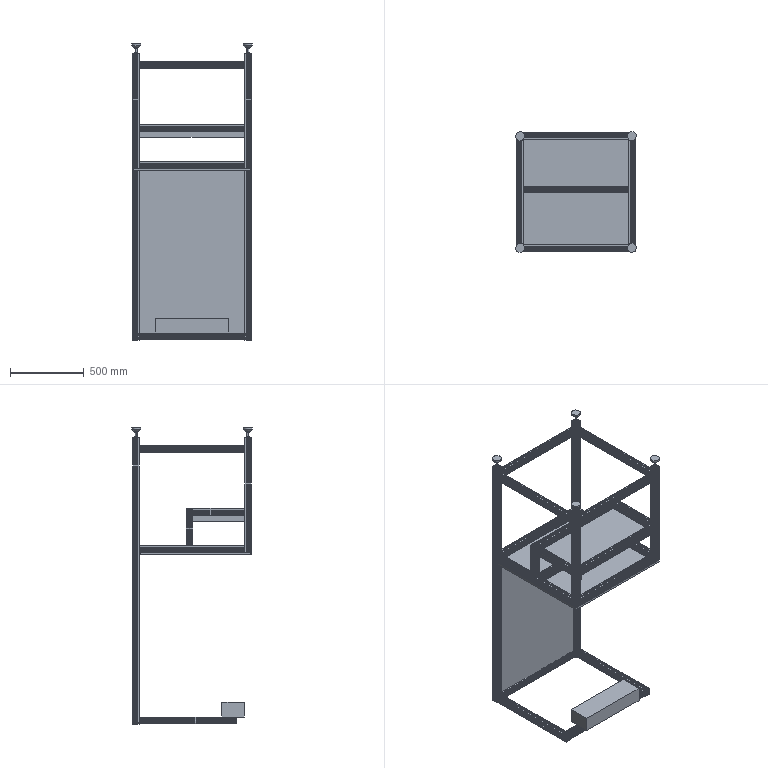Assembly | SolidWorks | mm | 41 component files | 41 solids | 3749 faces | box 815 x 815 x 2003 mm | volume 35568573 mm3 | plane 2366 | cylinder 1301 | cone 78 | spline 4 | commonest cylinder face diameters 2 x414 3 x276 1 x230 12.5 x145 6 x118 10 x36 2.5 x24 12 x16
Bill of materials:
dub02-B | 1 | Pine | Thin, nearly square flat plate with very small corner radii and no visible holes or other features.
FBR12nut | 4 |  | Hexagonal prism with a central round through-bore, with chamfered corners on both end faces. The shape is like a hex nut.
pad160_12_70pad1 | 4 |  | Part that turns around a single axis: a large circular disc with a short cylindrical rim and a conical taper underneath, a small hexagonal collar below the cone, and a long slender cylindrical shank with a chamfered end. The shape is like a leveling foot or swivel pad.
HFC8_4545_Bc | 6 |  | Square plate with rounded corners. A central cylindrical boss with a chamfered tip and several rectangular tabs stick out from its back face. It looks like a plug-in end cap.
HFS8_4545_01-B | 2 | 6061-T4 (SS) | Very long, slender straight prismatic bar with a constant square cross-section. Each of the four sides has one central undercut slot, there are four hollow corner pockets, and a central round bore with four small lobed holes around it. Ends are cut flat. This part is the most slender of the set.
HFS8_4545_02-B | 4 | 6061-T4 (SS) | Straight prismatic bar with a constant square cross-section. It has one undercut slot centred on each of its four sides, four hollow corner cavities, and a central round bore with four small lobed holes. Ends are cut flat.
HFS8_4545_03-B | 9 | 6061-T6 (SS) | Straight prismatic bar with a constant square cross-section. It has one undercut slot centred on each side, four corner cavities, and a central round bore with four small lobed holes. Ends are cut flat. The isometric view shows it in the mirrored orientation.
HFS8_4545_04-B | 2 |  | Long straight prismatic bar with a constant square cross-section. It has one undercut slot centred on each side, four corner cavities, and a central round bore with four small lobed holes. Ends are cut flat.
HFS8_4545_05-B | 2 |  | Straight prismatic bar with a constant square cross-section. It has one undercut slot centred on each of its four sides, four hollow corner cavities, and a central round bore with four small lobed holes. Ends are cut flat.
HFS8_4545_07-B | 2 |  | Short-to-medium straight prismatic bar with a constant square cross-section. It has one undercut slot centred on each side, four corner cavities, and a central round bore with four small lobed holes. Ends are cut flat.
HFS8_4545_08-B | 2 | 6061-T6 (SS) | Short straight prismatic bar with a constant square cross-section. It has one undercut slot centred on each of its four sides, four corner cavities, and a central round bore with four small lobed holes. Ends are cut flat. It is the shortest piece in the set.
HFS8_4545_09-B | 1 | Stainless Steel (Ferritic) | Thin rectangular sheet with short flanges bent downward along two opposite edges. This gives a shallow channel or cover shape.
ShadowlessLamp-B | 1 |  | Solid rectangular block (box shape) with sharp edges and no visible holes, chamfers, or cutouts.
V-GZT-0100-001 | 1 | Plexiglas (TM) GS Acrylic Cast Sheet | Very thin flat rectangular panel or sheet, taller than it is wide, with tiny corner radii and no visible features.
Mates:
1. coincident | HFS8_4545_01-B-1 face at (-85.006, -14.413, -2402.928) dir (0, -1, 0) | HFS8_4545_02-B-1 face at (-85.006, -14.413, -1239.928) dir (0, 1, 0)
2. coincident | HFS8_4545_01-B-1 face at (-43.006, -11.413, -2402.928) dir (1, 0, 0) | HFS8_4545_02-B-1 face at (-43.006, -14.413, -1239.928) dir (1, 0, 0)
3. coincident | HFS8_4545_01-B-1 face at (-88.006, 3.087, -2402.928) dir (-1, 0, 0) | HFS8_4545_03-B-1 face at (-88.006, -11.413, -1200.928) dir (1, 0, 0)
4. coincident | HFS8_4545_01-B-1 face at (-70.506, 30.587, -2402.928) dir (0, 1, 0) | HFS8_4545_03-B-1 face at (-798.006, 30.587, -1239.928) dir (0, 1, 0)
5. coincident | HFS8_4545_02-B-1 face at (-70.506, -14.413, -1197.928) dir (0, 0, 1) | HFS8_4545_03-B-1 face at (-798.006, 3.087, -1197.928) dir (0, 0, 1)
6. coincident | HFS8_4545_01-B-1 face at (-88.006, 3.087, -2402.928) dir (-1, 0, 0) | HFS8_4545_03-B-2 face at (-88.006, -11.413, -2360.928) dir (1, 0, 0)
7. coincident | HFS8_4545_01-B-1 face at (-85.006, -14.413, -2402.928) dir (0, -1, 0) | HFS8_4545_03-B-2 face at (-798.006, -14.413, -2385.428) dir (0, -1, 0)
8. coincident | HFS8_4545_01-B-1 face at (-85.006, -11.413, -2402.928) dir (0, 0, -1) | HFS8_4545_03-B-2 face at (-798.006, -11.413, -2402.928) dir (0, 0, -1)
9. coincident | HFS8_4545_01-B-1 face at (-85.006, -14.413, -2402.928) dir (0, -1, 0) | HFS8_4545_03-B-3 face at (-798.006, -14.413, -548.428) dir (0, -1, 0)
10. coincident | HFS8_4545_01-B-1 face at (-88.006, 27.587, -2402.928) dir (-1, 0, 0) | HFS8_4545_03-B-3 face at (-88.006, -11.413, -523.928) dir (1, 0, 0)
11. distance | HFS8_4545_03-B-3 face at (-798.006, 3.087, -520.928) dir (0, 0, 1) | HFS8_4545_01-B-1 face at (-85.006, -11.413, -470.928) dir (0, 0, 1)
12. coincident | HFS8_4545_01-B-2 face at (-815.506, -14.413, -2402.928) dir (0, -1, 0) | HFS8_4545_02-B-2 face at (-840.006, -14.413, -1239.928) dir (0, 1, 0)
13. coincident | HFS8_4545_01-B-2 face at (-843.006, 3.087, -2402.928) dir (-1, 0, 0) | HFS8_4545_02-B-2 face at (-843.006, -14.413, -1225.428) dir (-1, 0, 0)
14. coincident | HFS8_4545_03-B-1 face at (-798.006, 3.087, -1197.928) dir (0, 0, 1) | HFS8_4545_02-B-2 face at (-801.006, -14.413, -1197.928) dir (0, 0, 1)
15. coincident | HFS8_4545_01-B-2 face at (-815.506, -14.413, -2402.928) dir (0, -1, 0) | HFS8_4545_02-B-3 face at (-840.006, -14.413, -562.928) dir (0, 1, 0)
16. coincident | HFS8_4545_01-B-2 face at (-843.006, 3.087, -2402.928) dir (-1, 0, 0) | HFS8_4545_02-B-3 face at (-843.006, -14.413, -523.928) dir (-1, 0, 0)
17. coincident | HFS8_4545_03-B-3 face at (-798.006, 13.087, -565.928) dir (0, 0, -1) | HFS8_4545_02-B-3 face at (-815.506, -14.413, -565.928) dir (0, 0, -1)
18. coincident | HFS8_4545_02-B-4 edge at (-53.506, -14.413, -565.928) dir (0, -1, 0) | HFS8_4545_03-B-3 face at (-798.006, -11.413, -565.928) dir (0, 0, -1)
19. coincident | HFS8_4545_01-B-1 face at (-85.006, -14.413, -2402.928) dir (0, -1, 0) | HFS8_4545_02-B-4 face at (-85.006, -14.413, -564.928) dir (0, 1, 0)
20. coincident | HFS8_4545_01-B-1 face at (-43.006, -11.413, -2402.928) dir (1, 0, 0) | HFS8_4545_02-B-4 face at (-43.006, -14.413, -564.928) dir (1, 0, 0)
21. coincident | HFS8_4545_02-B-1 face at (-43.006, -14.413, -1239.928) dir (1, 0, 0) | HFS8_4545_04-B-1 face at (-43.006, -766.413, -1242.928) dir (1, 0, 0)
22. coincident | HFS8_4545_02-B-1 face at (-85.006, -724.413, -1239.928) dir (0, -1, 0) | HFS8_4545_04-B-1 face at (-46.006, -724.413, -1242.928) dir (0, 1, 0)
23. coincident | HFS8_4545_04-B-1 face at (-85.006, -769.413, -1242.928) dir (0, -1, 0) | HFS8_4545_04-B-2 face at (-840.006, -769.413, -1242.928) dir (0, -1, 0)
24. coincident | HFS8_4545_04-B-1 face at (-60.506, -769.413, -1242.928) dir (0, -1, 0) | HFS8_4545_04-B-2 face at (-815.506, -769.413, -1242.928) dir (0, -1, 0)
25. coincident | HFS8_4545_02-B-3 face at (-843.006, -14.413, -523.928) dir (-1, 0, 0) | HFS8_4545_04-B-2 face at (-843.006, -727.413, -1242.928) dir (-1, 0, 0)
26. coincident | HFS8_4545_04-B-1 face at (-88.006, -751.913, -1242.928) dir (-1, 0, 0) | HFS8_4545_03-B-4 face at (-88.006, -766.413, -525.928) dir (1, 0, 0)
27. coincident | HFS8_4545_04-B-1 face at (-85.006, -769.413, -1242.928) dir (0, -1, 0) | HFS8_4545_03-B-4 face at (-798.006, -769.413, -550.428) dir (0, -1, 0)
28. coincident | HFS8_4545_02-B-4 face at (-85.006, -14.413, -567.928) dir (0, 0, -1) | HFS8_4545_03-B-4 face at (-798.006, -741.913, -567.928) dir (0, 0, -1)
29. coincident | HFS8_4545_04-B-1 face at (-85.006, -769.413, -1242.928) dir (0, -1, 0) | HFS8_4545_03-B-5 face at (-798.006, -769.413, -1225.428) dir (0, -1, 0)
30. coincident | HFS8_4545_04-B-1 face at (-88.006, -727.413, -1242.928) dir (-1, 0, 0) | HFS8_4545_03-B-5 face at (-88.006, -766.413, -1200.928) dir (1, 0, 0)
31. coincident | HFS8_4545_04-B-1 face at (-85.006, -766.413, -1242.928) dir (0, 0, -1) | HFS8_4545_03-B-5 face at (-798.006, -766.413, -1242.928) dir (0, 0, -1)
32. coincident | HFS8_4545_01-B-1 face at (-60.506, -14.413, -2402.928) dir (0, -1, 0) | HFS8_4545_05-B-1 face at (-46.006, -14.413, -2360.928) dir (0, 1, 0)
33. coincident | HFS8_4545_01-B-1 face at (-43.006, -11.413, -2402.928) dir (1, 0, 0) | HFS8_4545_05-B-1 face at (-43.006, -14.413, -2399.928) dir (1, 0, 0)
34. coincident | HFS8_4545_01-B-1 face at (-85.006, -11.413, -2402.928) dir (0, 0, -1) | HFS8_4545_05-B-1 face at (-60.506, -14.413, -2402.928) dir (0, 0, -1)
35. coincident | HFS8_4545_01-B-2 face at (-840.006, -11.413, -2402.928) dir (0, 0, -1) | HFS8_4545_05-B-2 face at (-815.506, -14.413, -2402.928) dir (0, 0, -1)
36. coincident | HFS8_4545_01-B-2 face at (-840.006, -14.413, -2402.928) dir (0, -1, 0) | HFS8_4545_05-B-2 face at (-801.006, -14.413, -2360.928) dir (0, 1, 0)
37. coincident | HFS8_4545_05-B-1 face at (-85.006, -14.413, -2402.928) dir (0, 0, -1) | HFS8_4545_03-B-6 face at (-798.006, -641.913, -2402.928) dir (0, 0, -1)
38. coincident | HFS8_4545_05-B-1 face at (-46.006, -669.413, -2360.928) dir (0, -1, 0) | HFS8_4545_03-B-6 face at (-798.006, -669.413, -2385.428) dir (0, -1, 0)
39. coincident | HFS8_4545_02-B-1 face at (-88.006, -14.413, -1225.428) dir (-1, 0, 0) | HFS8_4545_03-B-7 face at (-88.006, -388.913, -1200.928) dir (1, 0, 0)
40. coincident | HFS8_4545_02-B-1 face at (-85.006, -14.413, -1242.928) dir (0, 0, -1) | HFS8_4545_03-B-7 face at (-798.006, -364.413, -1242.928) dir (0, 0, -1)
41. width | HFS8_4545_03-B-7 face at (-798.006, -346.913, -1239.928) dir (0, 1, 0) | HFS8_4545_03-B-7 face at (-798.006, -391.913, -1225.428) dir (0, -1, 0) | HFS8_4545_03-B-5 face at (-798.006, -724.413, -1239.928) dir (0, 1, 0) | HFS8_4545_03-B-1 face at (-798.006, -14.413, -1225.428) dir (0, -1, 0)
42. coincident | HFS8_4545_03-B-6 face at (-798.006, -651.913, -2357.928) dir (0, 0, 1) | ShadowlessLamp-B-1 face at (-693.006, -721.913, -2357.928) dir (0, 0, -1)
43. width | ShadowlessLamp-B-1 face at (-443.006, -571.913, -2307.928) dir (0, 1, 0) | ShadowlessLamp-B-1 face at (-443.006, -721.913, -2307.928) dir (0, -1, 0) | HFS8_4545_03-B-6 face at (-798.006, -669.413, -2385.428) dir (0, -1, 0) | HFS8_4545_03-B-6 face at (-798.006, -624.413, -2399.928) dir (0, 1, 0)
44. width | HFS8_4545_05-B-1 face at (-43.006, -14.413, -2399.928) dir (1, 0, 0) | HFS8_4545_05-B-2 face at (-843.006, -14.413, -2385.428) dir (-1, 0, 0) | ShadowlessLamp-B-1 face at (-193.006, -721.913, -2257.928) dir (1, 0, 0) | ShadowlessLamp-B-1 face at (-693.006, -721.913, -2257.928) dir (-1, 0, 0)
45. coincident | HFS8_4545_02-B-1 face at (-85.006, -14.413, -1242.928) dir (0, 0, -1) | dub02-B-1 face at (-443.006, -391.913, -1242.928) dir (0, 0, 1)
46. width | dub02-B-1 face at (-43.006, -14.413, -1257.928) dir (1, 0, 0) | dub02-B-1 face at (-843.006, -14.413, -1257.928) dir (-1, 0, 0) | HFS8_4545_02-B-2 face at (-843.006, -14.413, -1225.428) dir (-1, 0, 0) | HFS8_4545_02-B-1 face at (-43.006, -14.413, -1239.928) dir (1, 0, 0)
47. coincident | HFS8_4545_04-B-1 face at (-85.006, -769.413, -1242.928) dir (0, -1, 0) | dub02-B-1 face at (-43.006, -769.413, -1257.928) dir (0, -1, 0)
48. concentric | HFS8_4545_04-B-1 face at (-65.506, -746.913, -1242.928) dir (0, 0, 1) r 6.25 | FBR60_12_70-1/pad160_12_70pad1-1 face at (-65.506, -746.913, -402.928) dir (0, 0, -1) r 6
49. coincident | HFS8_4545_04-B-1 face at (-85.006, -766.413, -470.928) dir (0, 0, 1) | FBR60_12_70-1/FBR12nut-1 face at (-75.398, -741.248, -470.928) dir (0, 0, -1)
50. coincident | HFS8_4545_01-B-1 face at (-85.006, -11.413, -470.928) dir (0, 0, 1) | HFS8_4545_04-B-1 face at (-85.006, -766.413, -470.928) dir (0, 0, 1)
51. coincident | FBR60_12_70-2/pad160_12_70pad1-1 face at (-846.539, -732.005, -402.928) dir (0, 0, 1) | FBR60_12_70-3/pad160_12_70pad1-1 face at (-91.539, 22.995, -402.928) dir (0, 0, 1)
52. coincident | FBR60_12_70-2/pad160_12_70pad1-1 face at (-846.539, -732.005, -402.928) dir (0, 0, 1) | FBR60_12_70-4/pad160_12_70pad1-1 face at (-846.539, 22.995, -402.928) dir (0, 0, 1)
53. coincident | FBR60_12_70-1/pad160_12_70pad1-1 face at (-91.539, -732.005, -402.928) dir (0, 0, 1) | FBR60_12_70-2/pad160_12_70pad1-1 face at (-846.539, -732.005, -402.928) dir (0, 0, 1)
54. concentric | HFS8_4545_04-B-2 face at (-820.506, -746.913, -1242.928) dir (0, 0, 1) r 6.25 | FBR60_12_70-2/pad160_12_70pad1-1 face at (-820.506, -746.913, -402.928) dir (0, 0, -1) r 6
55. concentric | HFS8_4545_01-B-1 face at (-65.506, 8.087, -2402.928) dir (0, 0, 1) r 6.25 | FBR60_12_70-3/pad160_12_70pad1-1 face at (-65.506, 8.087, -402.928) dir (0, 0, -1) r 6
56. concentric | HFS8_4545_01-B-2 face at (-820.506, 8.087, -2402.928) dir (0, 0, 1) r 6.25 | FBR60_12_70-4/pad160_12_70pad1-1 face at (-820.506, 8.087, -402.928) dir (0, 0, -1) r 6
57. coincident | HFS8_4545_03-B-5 face at (-798.006, -741.913, -1242.928) dir (0, 0, -1) | dub02-B-1 face at (-443.006, -391.913, -1242.928) dir (0, 0, 1)
58. coincident | HFS8_4545_01-B-2 face at (-843.006, 3.087, -2402.928) dir (-1, 0, 0) | HFS8_4545_05-B-2 face at (-843.006, -14.413, -2385.428) dir (-1, 0, 0)
59. coincident | HFS8_4545_04-B-2 face at (-815.506, -769.413, -1242.928) dir (0, -1, 0) | HFS8_4545_03-B-9 face at (-798.006, -769.413, -950.928) dir (0, -1, 0)
60. coincident | HFS8_4545_04-B-2 face at (-798.006, -766.413, -1242.928) dir (1, 0, 0) | HFS8_4545_03-B-9 face at (-798.006, -766.413, -950.928) dir (-1, 0, 0)
61. coincident | HFS8_4545_04-B-1 face at (-70.506, -724.413, -1242.928) dir (0, 1, 0) | HFS8_4545_07-B-1 face at (-85.006, -724.413, -989.928) dir (0, -1, 0)
62. coincident | HFS8_4545_04-B-1 face at (-43.006, -741.913, -1242.928) dir (1, 0, 0) | HFS8_4545_07-B-1 face at (-43.006, -374.413, -989.928) dir (1, 0, 0)
63. coincident | HFS8_4545_07-B-1 face at (-60.506, -374.413, -992.928) dir (0, 0, -1) | HFS8_4545_03-B-9 face at (-798.006, -741.913, -992.928) dir (0, 0, -1)
64. coincident | HFS8_4545_08-B-3 face at (-70.506, -329.413, -1197.928) dir (0, 1, 0) | HFS8_4545_03-B-11 face at (-798.006, -329.413, -989.928) dir (0, 1, 0)
65. coincident | HFS8_4545_08-B-3 face at (-85.006, -371.413, -947.928) dir (0, 0, 1) | HFS8_4545_03-B-11 face at (-798.006, -332.413, -947.928) dir (0, 0, 1)
66. coincident | HFS8_4545_07-B-3 face at (-815.506, -374.413, -992.928) dir (0, 0, -1) | HFS8_4545_03-B-11 face at (-798.006, -346.913, -992.928) dir (0, 0, -1)
67. coincident | HFS8_4545_07-B-3 face at (-843.006, -374.413, -975.428) dir (-1, 0, 0) | HFS8_4545_08-B-4 face at (-843.006, -356.913, -1197.928) dir (-1, 0, 0)
68. coincident | HFS8_4545_07-B-3 face at (-840.006, -374.413, -989.928) dir (0, 1, 0) | HFS8_4545_08-B-4 face at (-840.006, -374.413, -1197.928) dir (0, -1, 0)
69. coincident | HFS8_4545_03-B-11 face at (-798.006, -329.413, -989.928) dir (0, 1, 0) | HFS8_4545_09-B-2 face at (-443.006, -329.413, -994.928) dir (0, 1, 0)
70. coincident | HFS8_4545_02-B-1 face at (-70.506, -14.413, -1197.928) dir (0, 0, 1) | HFS8_4545_08-B-3 face at (-85.006, -371.413, -1197.928) dir (0, 0, -1)
71. coincident | HFS8_4545_07-B-1 face at (-43.006, -374.413, -989.928) dir (1, 0, 0) | HFS8_4545_08-B-3 face at (-43.006, -346.913, -1197.928) dir (1, 0, 0)
72. coincident | HFS8_4545_07-B-1 face at (-85.006, -374.413, -989.928) dir (0, 1, 0) | HFS8_4545_08-B-3 face at (-85.006, -374.413, -1197.928) dir (0, -1, 0)
73. coincident | HFS8_4545_04-B-2 face at (-801.006, -724.413, -1242.928) dir (0, 1, 0) | HFS8_4545_07-B-3 face at (-840.006, -724.413, -989.928) dir (0, -1, 0)
74. coincident | HFS8_4545_03-B-9 face at (-798.006, -741.913, -992.928) dir (0, 0, -1) | HFS8_4545_07-B-3 face at (-840.006, -374.413, -992.928) dir (0, 0, -1)
75. coincident | HFS8_4545_04-B-2 face at (-843.006, -727.413, -1242.928) dir (-1, 0, 0) | HFS8_4545_07-B-3 face at (-843.006, -374.413, -950.928) dir (-1, 0, 0)
76. coincident | HFS8_4545_07-B-1 face at (-88.006, -374.413, -975.428) dir (-1, 0, 0) | HFS8_4545_03-B-11 face at (-88.006, -371.413, -950.928) dir (1, 0, 0)
77. coincident | HFS8_4545_02-B-2 face at (-801.006, -14.413, -1197.928) dir (0, 0, 1) | HFS8_4545_08-B-4 face at (-840.006, -371.413, -1197.928) dir (0, 0, -1)
78. coincident | HFS8_4545_03-B-9 face at (-798.006, -741.913, -992.928) dir (0, 0, -1) | HFS8_4545_09-B-2 face at (-443.006, -551.413, -992.928) dir (0, 0, 1)
79. coincident | HFS8_4545_04-B-2 face at (-798.006, -741.913, -1242.928) dir (1, 0, 0) | HFS8_4545_09-B-2 face at (-798.006, -551.413, -994.928) dir (-1, 0, 0)
80. coincident | HFS8_4545_05-B-2 face at (-801.006, -669.413, -2360.928) dir (0, -1, 0) | HFC8_4545_B-1/HFC8_4545_Bc-1 face at (-840.006, -669.413, -2399.928) dir (0, 1, 0)
81. width | HFC8_4545_B-1/HFC8_4545_Bc-1 face at (-840.006, -672.413, -2357.928) dir (0, 0, 1) | HFC8_4545_B-1/HFC8_4545_Bc-1 face at (-801.006, -672.413, -2402.928) dir (0, 0, -1) | HFS8_4545_05-B-2 face at (-840.006, -14.413, -2402.928) dir (0, 0, -1) | HFS8_4545_05-B-2 face at (-825.506, -14.413, -2357.928) dir (0, 0, 1)
82. width | HFS8_4545_05-B-2 face at (-798.006, -14.413, -2375.428) dir (1, 0, 0) | HFS8_4545_05-B-2 face at (-843.006, -14.413, -2360.928) dir (-1, 0, 0) | HFC8_4545_B-1/HFC8_4545_Bc-1 face at (-843.006, -672.413, -2399.928) dir (-1, 0, 0) | HFC8_4545_B-1/HFC8_4545_Bc-1 face at (-798.006, -672.413, -2360.928) dir (1, 0, 0)
83. coincident | HFS8_4545_05-B-1 face at (-88.006, -14.413, -2385.428) dir (-1, 0, 0) | HFS8_4545_03-B-6 face at (-88.006, -666.413, -2360.928) dir (1, 0, 0)
84. coincident | HFC8_4545_B-1/HFC8_4545_Bc-1 face at (-840.006, -672.413, -2399.928) dir (0, -1, 0) | HFC8_4545_Bc-1 face at (-46.006, -672.413, -2360.928) dir (0, -1, 0)
85. coincident | HFC8_4545_B-1/HFC8_4545_Bc-1 face at (-801.006, -672.413, -2402.928) dir (0, 0, -1) | HFC8_4545_Bc-1 face at (-46.006, -672.413, -2402.928) dir (0, 0, -1)
86. coincident | HFS8_4545_05-B-1 face at (-43.006, -14.413, -2399.928) dir (1, 0, 0) | HFC8_4545_Bc-1 face at (-43.006, -672.413, -2360.928) dir (1, 0, 0)
87. coincident | HFC8_4545_Bc-2 face at (-46.006, -332.413, -944.928) dir (0, 0, 1) | HFC8_4545_Bc-3 face at (-801.006, -332.413, -944.928) dir (0, 0, 1)
88. coincident | HFS8_4545_08-B-3 face at (-85.006, -371.413, -947.928) dir (0, 0, 1) | HFC8_4545_Bc-2 face at (-46.006, -332.413, -947.928) dir (0, 0, -1)
89. coincident | HFS8_4545_08-B-3 face at (-43.006, -346.913, -1197.928) dir (1, 0, 0) | HFC8_4545_Bc-2 face at (-43.006, -332.413, -944.928) dir (1, 0, 0)
90. coincident | HFS8_4545_08-B-3 face at (-46.006, -329.413, -1197.928) dir (0, 1, 0) | HFC8_4545_Bc-2 face at (-85.006, -329.413, -944.928) dir (0, 1, 0)
91. coincident | HFS8_4545_08-B-4 face at (-843.006, -356.913, -1197.928) dir (-1, 0, 0) | HFC8_4545_Bc-3 face at (-843.006, -371.413, -944.928) dir (-1, 0, 0)
92. coincident | HFS8_4545_08-B-4 face at (-825.506, -329.413, -1197.928) dir (0, 1, 0) | HFC8_4545_Bc-3 face at (-840.006, -329.413, -944.928) dir (0, 1, 0)
93. width | V-GZT-0100-001-1 face at (-810.506, 5.587, -2370.428) dir (0, 0, -1) | V-GZT-0100-001-1 face at (-810.506, 5.587, -1230.428) dir (0, 0, 1) | HFS8_4545_03-B-2 face at (-798.006, 27.587, -2357.928) dir (0, 0, 1) | HFS8_4545_03-B-1 face at (-798.006, 13.087, -1242.928) dir (0, 0, -1)
94. width | HFS8_4545_01-B-2 face at (-843.006, 27.587, -2402.928) dir (-1, 0, 0) | HFS8_4545_01-B-1 face at (-43.006, 13.087, -2402.928) dir (1, 0, 0) | V-GZT-0100-001-1 face at (-810.506, 5.587, -2370.428) dir (-1, 0, 0) | V-GZT-0100-001-1 face at (-75.506, 5.587, -2370.428) dir (1, 0, 0)
95. width | V-GZT-0100-001-1 face at (-443.006, 5.587, -1800.428) dir (0, -1, 0) | V-GZT-0100-001-1 face at (-443.006, 10.587, -1800.428) dir (0, 1, 0) | HFS8_4545_01-B-2 face at (-815.506, -14.413, -2402.928) dir (0, -1, 0) | HFS8_4545_01-B-2 face at (-801.006, 30.587, -2402.928) dir (0, 1, 0)
96. coincident | HFC8_4545_B-2/HFC8_4545_Bc-1 face at (-85.006, 27.587, -2405.928) dir (0, 0, -1) | HFC8_4545_Bc-4 face at (-840.006, 27.587, -2405.928) dir (0, 0, -1)
97. coincident | HFC8_4545_B-2/HFC8_4545_Bc-1 face at (-46.006, 30.587, -2405.928) dir (0, 1, 0) | HFC8_4545_Bc-4 face at (-801.006, 30.587, -2405.928) dir (0, 1, 0)
98. coincident | HFS8_4545_01-B-1 face at (-85.006, -11.413, -2402.928) dir (0, 0, -1) | HFC8_4545_Bc-4 face at (-840.006, 27.587, -2402.928) dir (0, 0, 1)
99. coincident | HFS8_4545_01-B-1 face at (-46.006, 30.587, -2402.928) dir (0, 1, 0) | HFC8_4545_B-2/HFC8_4545_Bc-1 face at (-46.006, 30.587, -2405.928) dir (0, 1, 0)
100. coincident | HFS8_4545_01-B-1 face at (-43.006, 13.087, -2402.928) dir (1, 0, 0) | HFC8_4545_B-2/HFC8_4545_Bc-1 face at (-43.006, -11.413, -2405.928) dir (1, 0, 0)
101. coincident | HFS8_4545_01-B-2 face at (-843.006, 27.587, -2402.928) dir (-1, 0, 0) | HFC8_4545_Bc-4 face at (-843.006, 27.587, -2405.928) dir (-1, 0, 0)
102. coincident | pad160_12_70pad1-1 axis at (0, 50, 0) dir (0, -1, 0) | FBR12nut-1 axis at (0, 18, 0) dir (0, 1, 0)